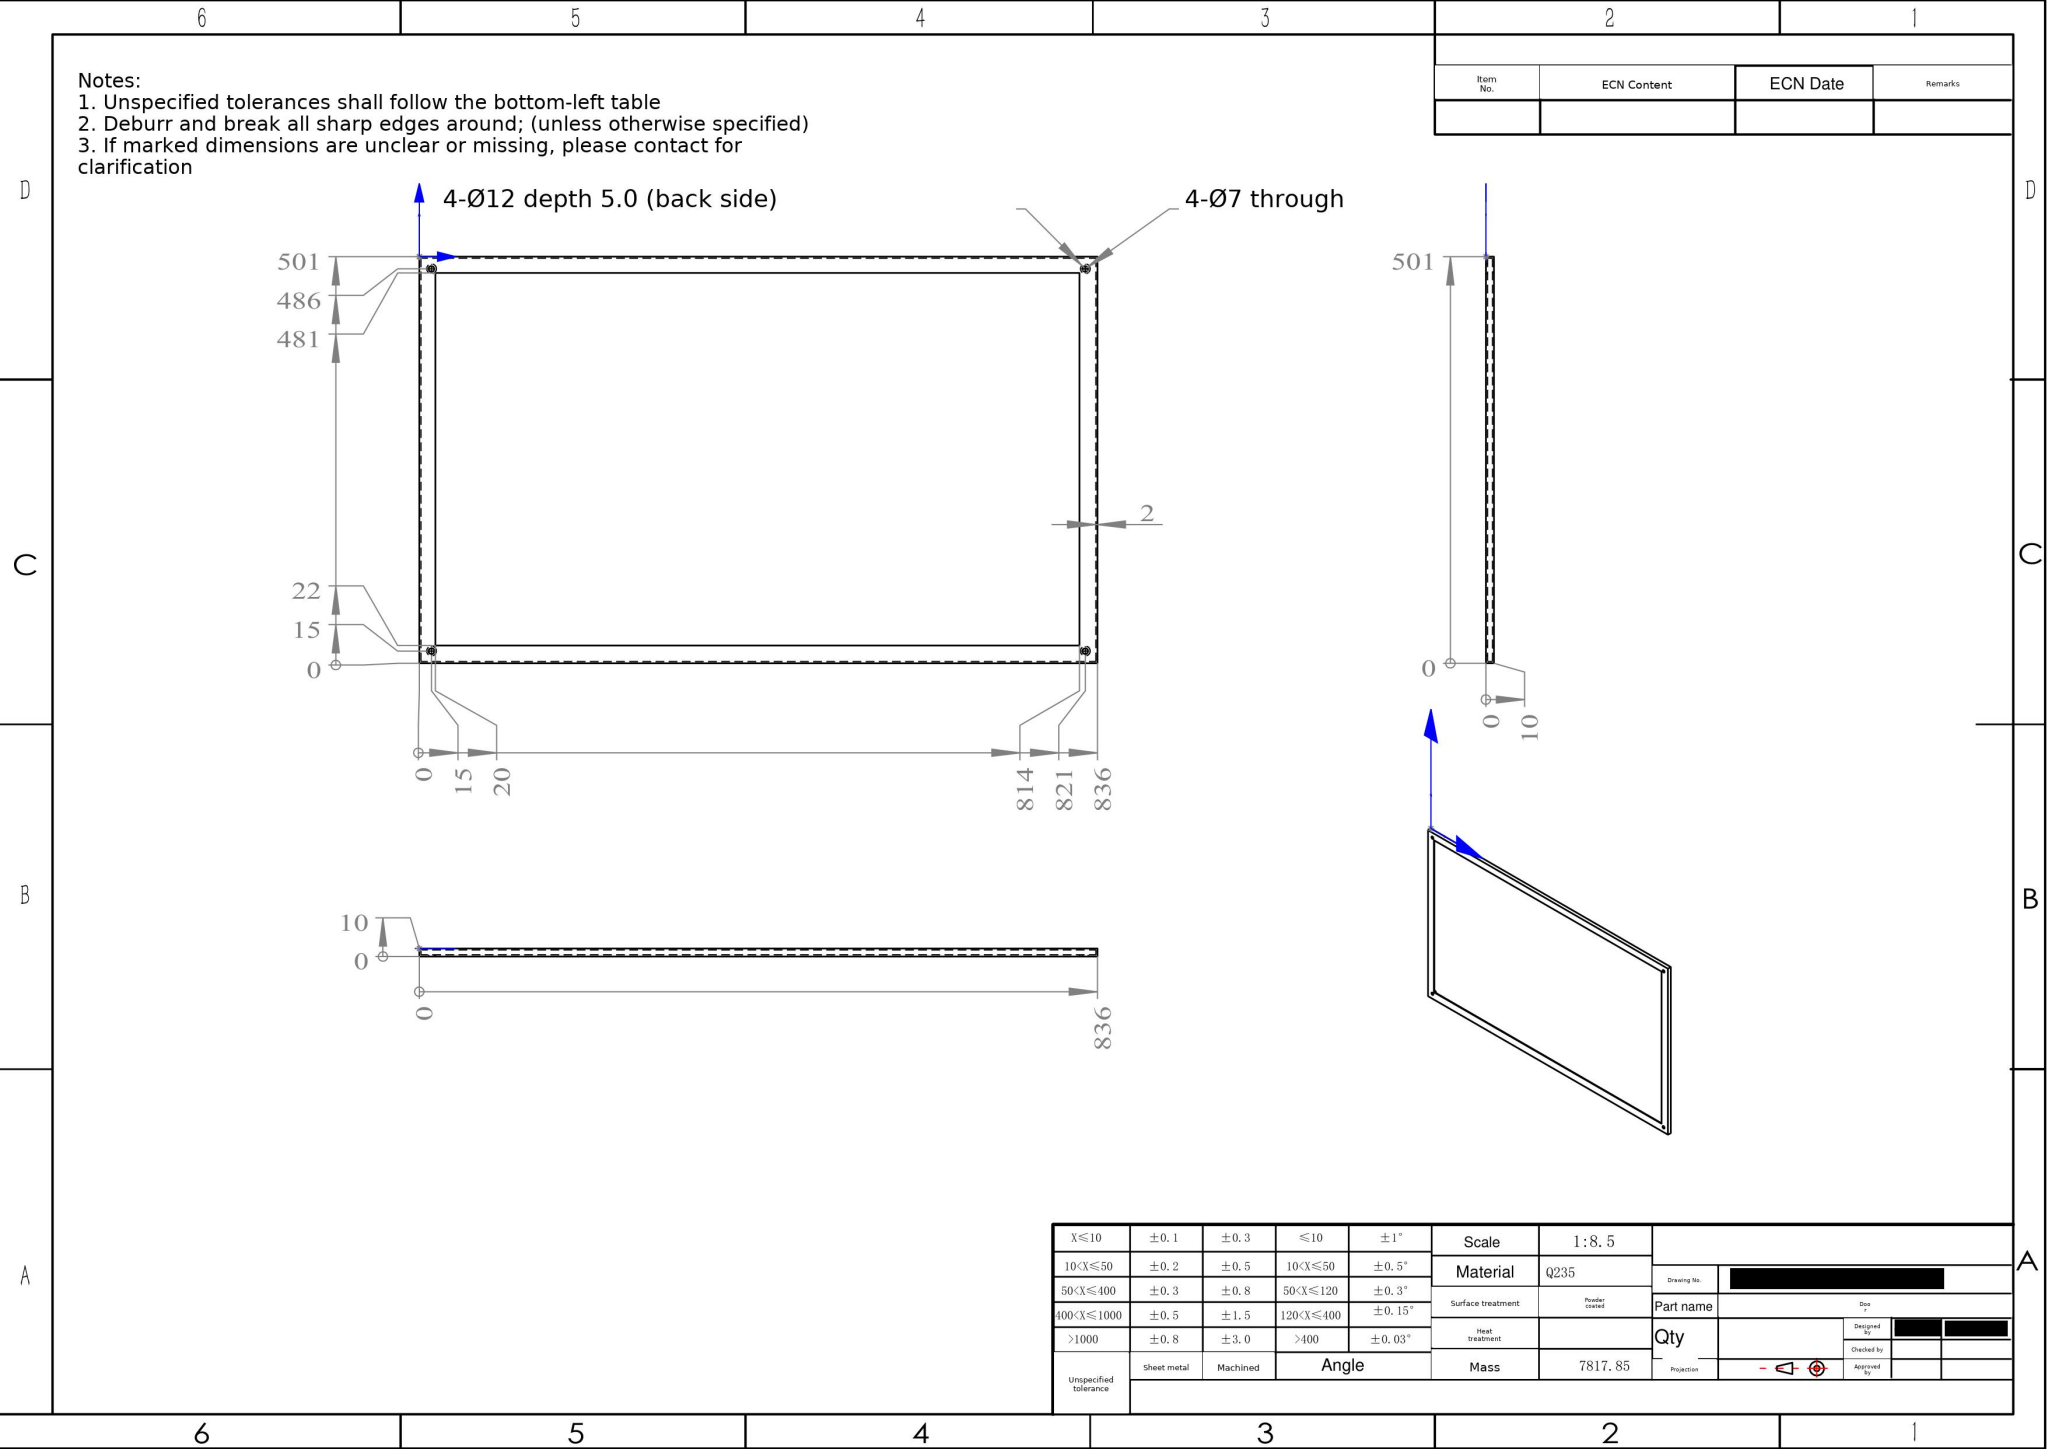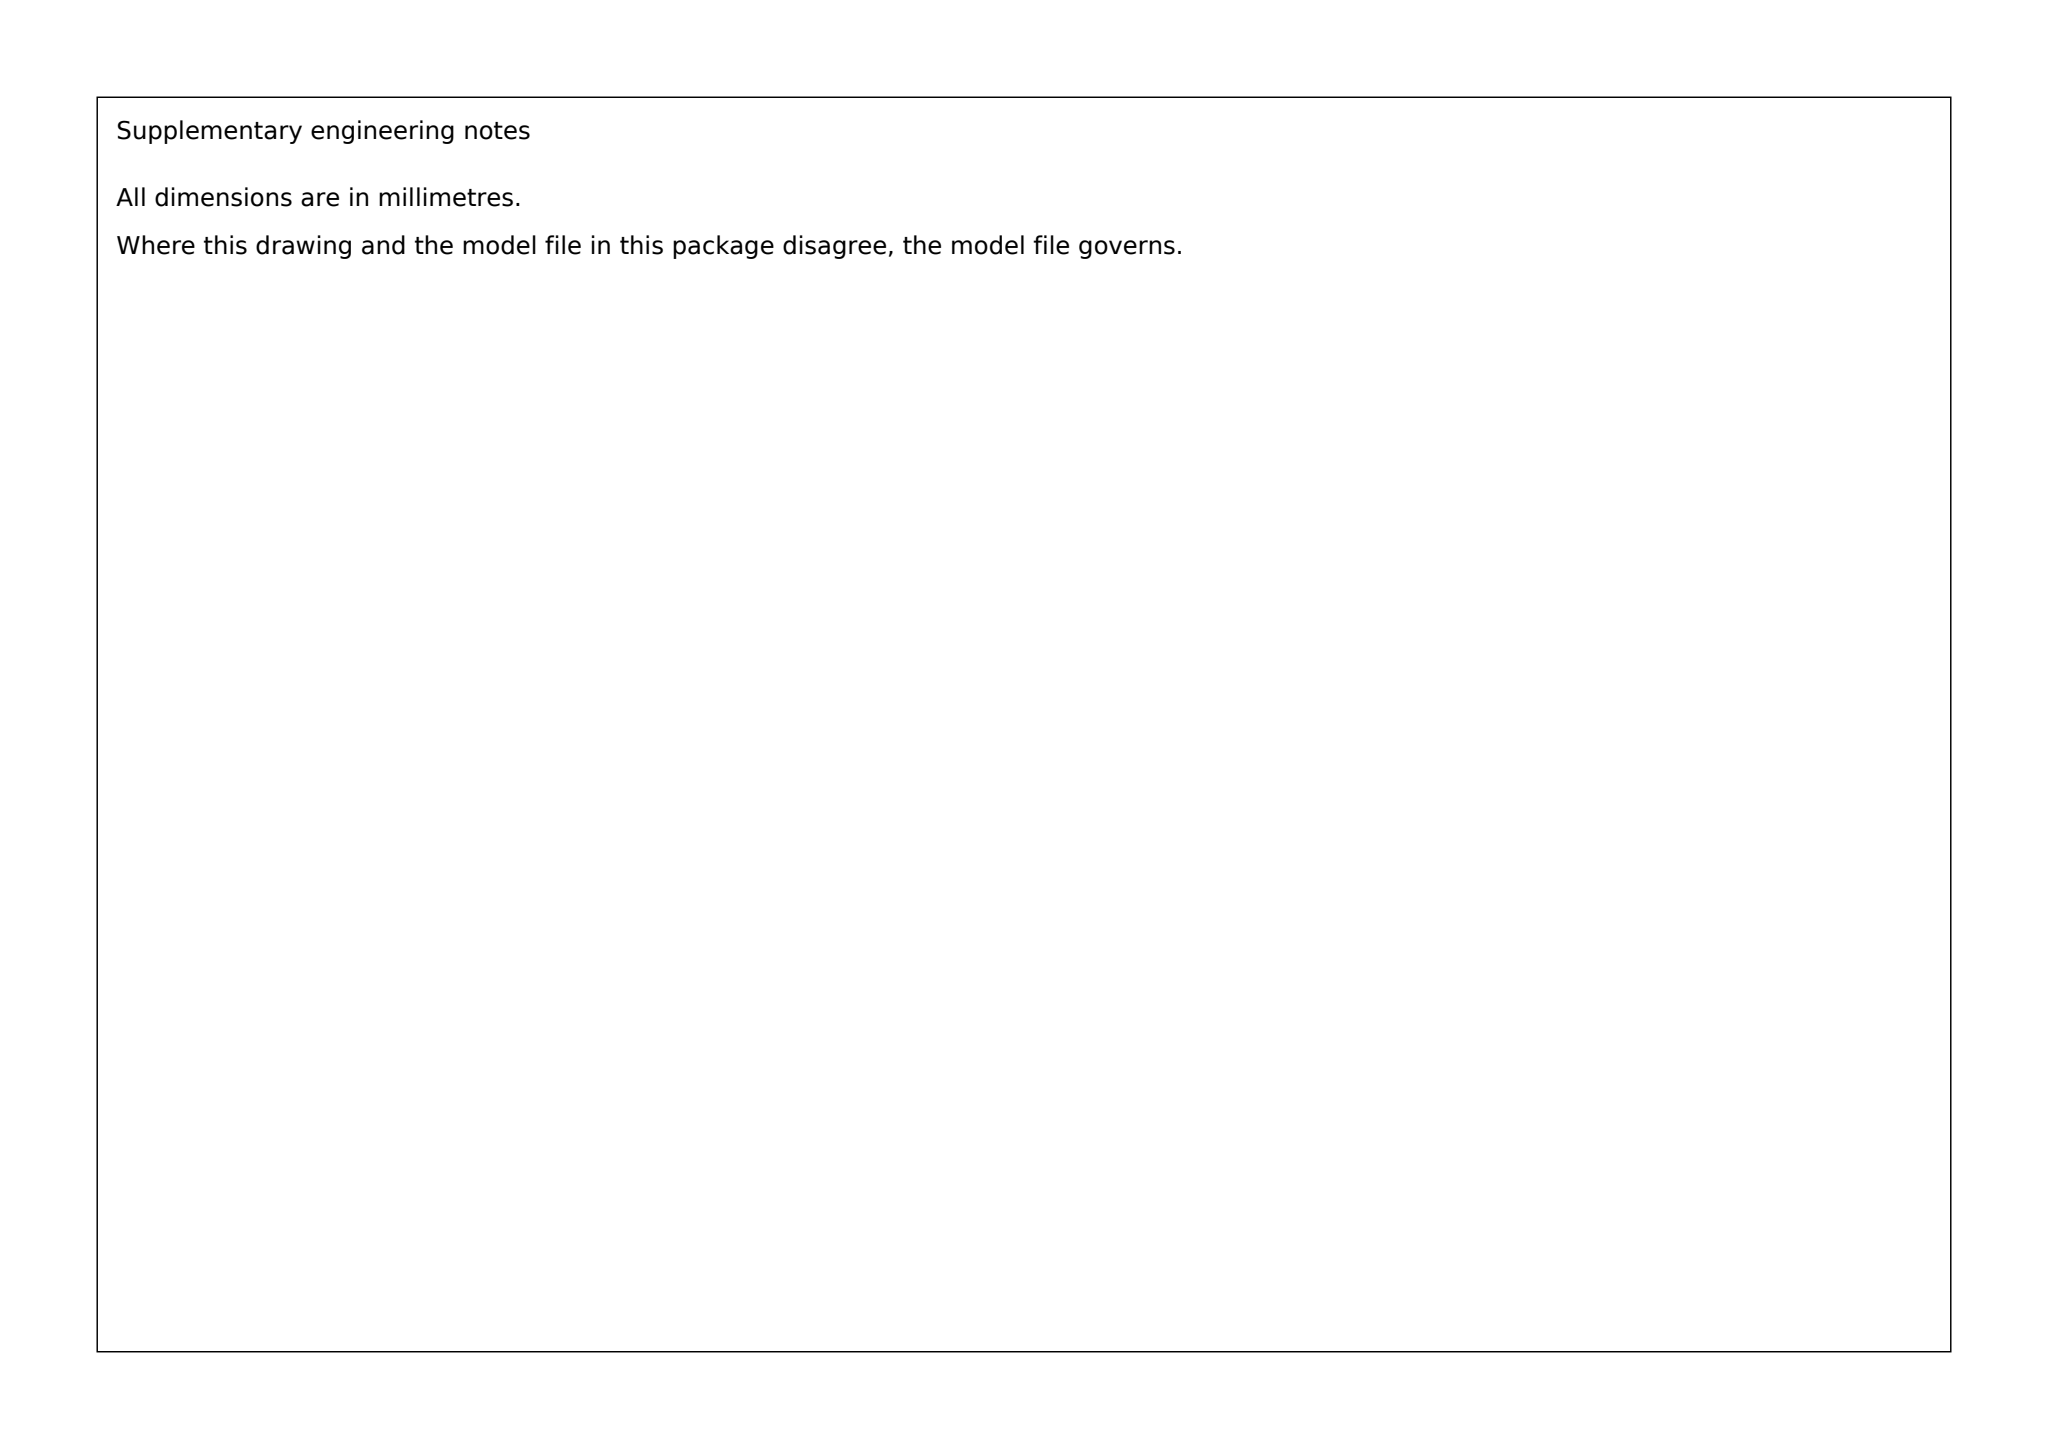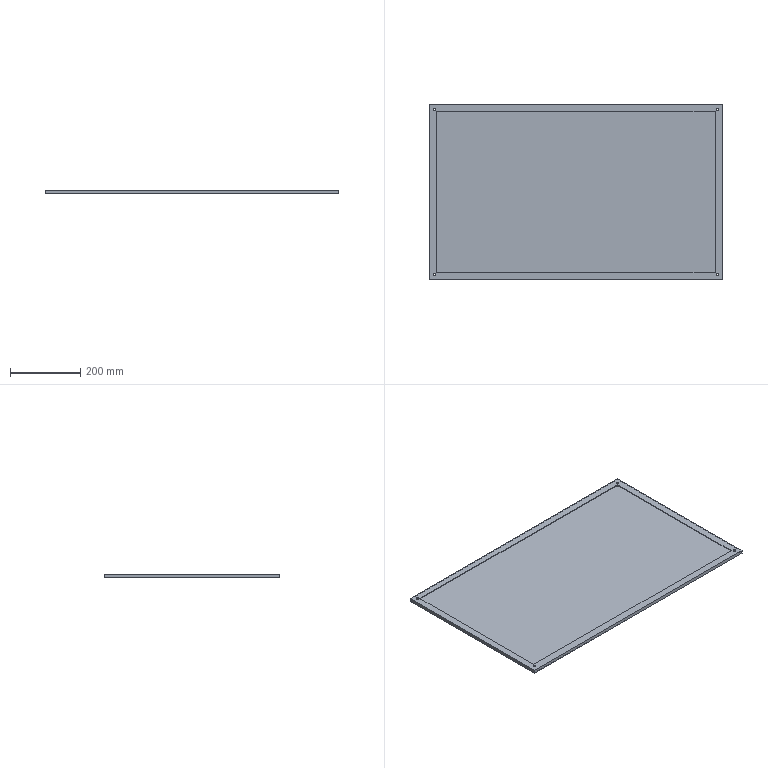Part | SolidWorks | mm | material Q235 | 1 solid | 32 faces | box 836 x 501 x 10 mm | volume 977231 mm3 | cylinder 16 | plane 16 | commonest cylinder face diameters 7 x8 12 x8
build123d program:
from build123d import *

# Parameters (mm, degrees)
SKETCH1_W           = 836
SKETCH1_H           = 501
BOSS_EXTRUDE1_DEPTH = 10
SHELL1_T            = -2
SKETCH2_W           = 836
SKETCH2_H           = 501
SKETCH2_W_2         = 794
SKETCH2_H_2         = 459
BOSS_EXTRUDE2_DEPTH = 2
SKETCH3_R           = 6
CUT_EXTRUDE1_DEPTH  = 5
SKETCH4_R           = 3.5
CUT_EXTRUDE2_DEPTH  = 975.678


with BuildPart() as part:
    # Sketch1 → Boss-Extrude1 (new body)
    with BuildSketch(Plane.XY):
        with Locations((418, -250.5)):
            Rectangle(SKETCH1_W, SKETCH1_H)
    extrude(amount=BOSS_EXTRUDE1_DEPTH)

    # Shell1
    shell1_openings = [part.faces().sort_by_distance(p)[0] for p in [
        (418, -250.5, 10),
    ]]
    offset(amount=SHELL1_T, openings=shell1_openings, kind=Kind.INTERSECTION)

    # Sketch2 → Boss-Extrude2 (add)
    with BuildSketch(Plane.XY.offset(10)):
        with Locations((418, -250.5)):
            Rectangle(SKETCH2_W, SKETCH2_H)
        with Locations((417, -249.5)):
            Rectangle(SKETCH2_W_2, SKETCH2_H_2, mode=Mode.SUBTRACT)
    extrude(amount=-BOSS_EXTRUDE2_DEPTH)

    # Sketch3 → Cut-Extrude1 (cut)
    with BuildSketch(Plane(origin=(0, 0, 0), x_dir=(-1, 0, 0), z_dir=(0, 0, -1))):
        with Locations((-821, -15)):
            Circle(SKETCH3_R)
        with Locations((-15, -15)):
            Circle(SKETCH3_R)
        with Locations((-821, -486)):
            Circle(SKETCH3_R)
        with Locations((-15, -486)):
            Circle(SKETCH3_R)
    extrude(amount=-CUT_EXTRUDE1_DEPTH, mode=Mode.SUBTRACT)

    # Sketch4 → Cut-Extrude2 (cut, through all)
    with BuildSketch(Plane(origin=(0, 0, 0), x_dir=(-1, 0, 0), z_dir=(0, 0, -1))):
        with Locations((-821, -15)):
            Circle(SKETCH4_R)
        with Locations((-15, -15)):
            Circle(SKETCH4_R)
        with Locations((-15, -486)):
            Circle(SKETCH4_R)
        with Locations((-821, -486)):
            Circle(SKETCH4_R)
    extrude(amount=-CUT_EXTRUDE2_DEPTH, mode=Mode.SUBTRACT)


solid = part.part